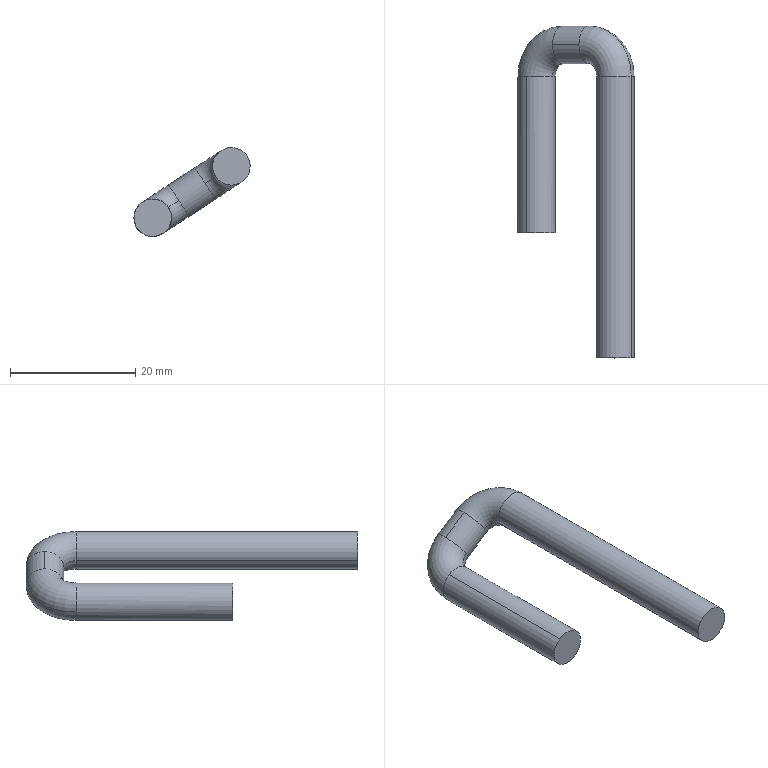Component | SolidWorks | 75-02-24RotatingHook-1 | 1 solid | 12 faces | box 18.56 x 53 x 14.2 mm | volume 2565 mm3 | cylinder 6 | torus 4 | plane 2 | commonest cylinder face diameters 6 x6 | material A3 Steel
build123d program:
from build123d import *

# Parameters (mm, degrees)
SWEEP1_PROFILE_R = 3


with BuildPart() as part:
    # Sweep1: sweep along a path in Sketch1
    with BuildLine(Plane.XY) as sweep1_path:
        Line((0, 50), (0, 5))
        ThreePointArc((0, 5), (1.464, 1.464), (5, 0))
        Line((5, 0), (10, 0))
        ThreePointArc((10, 0), (13.536, 1.464), (15, 5))
        Line((15, 5), (15, 30))
    # Sweep1 profile (on start of the path) → Sweep1 (sweep)
    with BuildSketch(Plane(origin=(0, 50, 0), x_dir=(-1, 0, 0), z_dir=(0, -1, 0))):
        Circle(SWEEP1_PROFILE_R)
    sweep(path=sweep1_path.line)


solid = part.part

# Placed as in the assembly
solid = solid.moved(Location((-17.87, 315.857, -43.68), (0, -33.158, -180)))
STEP:
#1=COLOUR_RGB('',0.7922,0.8196,0.9333);
#2=FILL_AREA_STYLE_COLOUR('',#1);
#3=FILL_AREA_STYLE('',(#2));
#4=SURFACE_STYLE_FILL_AREA(#3);
#5=SURFACE_SIDE_STYLE('',(#4));
#6=SURFACE_STYLE_USAGE(.BOTH.,#5);
#7=PRESENTATION_STYLE_ASSIGNMENT((#6));
#8=CARTESIAN_POINT('',(-1.033,12.553,-1.935));
#9=VERTEX_POINT('',#8);
#10=CARTESIAN_POINT('',(-1.098,12.435,-1.836));
#11=VERTEX_POINT('',#10);
#12=CARTESIAN_POINT('',(-1.033,12.435,-1.935));
#13=DIRECTION('',(0.8372,-0.,0.5469));
#14=DIRECTION('',(0.5469,0.,-0.8372));
#15=AXIS2_PLACEMENT_3D('',#12,#13,#14);
#16=CIRCLE('',#15,0.1181);
#17=EDGE_CURVE('',#9,#11,#16,.T.);
#18=ORIENTED_EDGE('',*,*,#17,.F.);
#19=CARTESIAN_POINT('',(-1.297,12.238,-2.107));
#20=VERTEX_POINT('',#19);
#21=CARTESIAN_POINT('',(-1.033,12.238,-1.935));
#22=DIRECTION('',(-0.5469,-0.,0.8372));
#23=DIRECTION('',(0.8372,0.,0.5469));
#24=AXIS2_PLACEMENT_3D('',#21,#22,#23);
#25=CIRCLE('',#24,0.315);
#26=EDGE_CURVE('',#9,#20,#25,.T.);
#27=ORIENTED_EDGE('',*,*,#26,.T.);
#28=CARTESIAN_POINT('',(-1.263,12.238,-1.944));
#29=VERTEX_POINT('',#28);
#30=CARTESIAN_POINT('',(-1.198,12.238,-2.043));
#31=DIRECTION('',(-0.,1.,0.));
#32=DIRECTION('',(0.5469,0.,-0.8372));
#33=AXIS2_PLACEMENT_3D('',#30,#31,#32);
#34=CIRCLE('',#33,0.1181);
#35=EDGE_CURVE('',#20,#29,#34,.T.);
#36=ORIENTED_EDGE('',*,*,#35,.T.);
#37=CARTESIAN_POINT('',(-1.099,12.238,-1.978));
#38=VERTEX_POINT('',#37);
#39=CARTESIAN_POINT('',(-1.198,12.238,-2.043));
#40=DIRECTION('',(-0.,1.,0.));
#41=DIRECTION('',(0.5469,0.,-0.8372));
#42=AXIS2_PLACEMENT_3D('',#39,#40,#41);
#43=CIRCLE('',#42,0.1181);
#44=EDGE_CURVE('',#29,#38,#43,.T.);
#45=ORIENTED_EDGE('',*,*,#44,.T.);
#46=CARTESIAN_POINT('',(-1.033,12.317,-1.935));
#47=VERTEX_POINT('',#46);
#48=CARTESIAN_POINT('',(-1.033,12.238,-1.935));
#49=DIRECTION('',(-0.5469,-0.,0.8372));
#50=DIRECTION('',(0.8372,0.,0.5469));
#51=AXIS2_PLACEMENT_3D('',#48,#49,#50);
#52=CIRCLE('',#51,0.07874);
#53=EDGE_CURVE('',#47,#38,#52,.T.);
#54=ORIENTED_EDGE('',*,*,#53,.F.);
#55=CARTESIAN_POINT('',(-1.033,12.435,-1.935));
#56=DIRECTION('',(0.8372,-0.,0.5469));
#57=DIRECTION('',(0.5469,0.,-0.8372));
#58=AXIS2_PLACEMENT_3D('',#55,#56,#57);
#59=CIRCLE('',#58,0.1181);
#60=EDGE_CURVE('',#11,#47,#59,.T.);
#61=ORIENTED_EDGE('',*,*,#60,.F.);
#62=EDGE_LOOP('',(#18,#27,#36,#45,#54,#61));
#63=FACE_OUTER_BOUND('',#62,.T.);
#64=CARTESIAN_POINT('',(-1.033,12.238,-1.935));
#65=DIRECTION('',(-0.5469,-0.,0.8372));
#66=DIRECTION('',(-0.8372,0.,-0.5469));
#67=AXIS2_PLACEMENT_3D('',#64,#65,#66);
#68=TOROIDAL_SURFACE('',#67,0.1969,0.1181);
#69=ADVANCED_FACE('',(#63),#68,.T.);
#70=CARTESIAN_POINT('',(-0.6047,12.238,-1.655));
#71=VERTEX_POINT('',#70);
#72=CARTESIAN_POINT('',(-0.8024,12.238,-1.784));
#73=VERTEX_POINT('',#72);
#74=CARTESIAN_POINT('',(-0.7036,12.238,-1.72));
#75=DIRECTION('',(-0.,-1.,-0.));
#76=DIRECTION('',(0.5469,0.,-0.8372));
#77=AXIS2_PLACEMENT_3D('',#74,#75,#76);
#78=CIRCLE('',#77,0.1181);
#79=EDGE_CURVE('',#71,#73,#78,.T.);
#80=ORIENTED_EDGE('',*,*,#79,.F.);
#81=CARTESIAN_POINT('',(-0.8684,12.553,-1.827));
#82=VERTEX_POINT('',#81);
#83=CARTESIAN_POINT('',(-0.8684,12.238,-1.827));
#84=DIRECTION('',(-0.5469,-0.,0.8372));
#85=DIRECTION('',(0.8372,0.,0.5469));
#86=AXIS2_PLACEMENT_3D('',#83,#84,#85);
#87=CIRCLE('',#86,0.315);
#88=EDGE_CURVE('',#71,#82,#87,.T.);
#89=ORIENTED_EDGE('',*,*,#88,.T.);
#90=CARTESIAN_POINT('',(-0.933,12.435,-1.728));
#91=VERTEX_POINT('',#90);
#92=CARTESIAN_POINT('',(-0.8684,12.435,-1.827));
#93=DIRECTION('',(0.8372,0.,0.5469));
#94=DIRECTION('',(0.5469,0.,-0.8372));
#95=AXIS2_PLACEMENT_3D('',#92,#93,#94);
#96=CIRCLE('',#95,0.1181);
#97=EDGE_CURVE('',#82,#91,#96,.T.);
#98=ORIENTED_EDGE('',*,*,#97,.T.);
#99=CARTESIAN_POINT('',(-0.8684,12.317,-1.827));
#100=VERTEX_POINT('',#99);
#101=CARTESIAN_POINT('',(-0.8684,12.435,-1.827));
#102=DIRECTION('',(0.8372,0.,0.5469));
#103=DIRECTION('',(0.5469,0.,-0.8372));
#104=AXIS2_PLACEMENT_3D('',#101,#102,#103);
#105=CIRCLE('',#104,0.1181);
#106=EDGE_CURVE('',#91,#100,#105,.T.);
#107=ORIENTED_EDGE('',*,*,#106,.T.);
#108=CARTESIAN_POINT('',(-0.8684,12.238,-1.827));
#109=DIRECTION('',(-0.5469,-0.,0.8372));
#110=DIRECTION('',(0.8372,0.,0.5469));
#111=AXIS2_PLACEMENT_3D('',#108,#109,#110);
#112=CIRCLE('',#111,0.07874);
#113=EDGE_CURVE('',#73,#100,#112,.T.);
#114=ORIENTED_EDGE('',*,*,#113,.F.);
#115=EDGE_LOOP('',(#80,#89,#98,#107,#114));
#116=FACE_OUTER_BOUND('',#115,.T.);
#117=CARTESIAN_POINT('',(-0.8684,12.238,-1.827));
#118=DIRECTION('',(-0.5469,-0.,0.8372));
#119=DIRECTION('',(-0.8372,0.,-0.5469));
#120=AXIS2_PLACEMENT_3D('',#117,#118,#119);
#121=TOROIDAL_SURFACE('',#120,0.1969,0.1181);
#122=ADVANCED_FACE('',(#116),#121,.T.);
#123=CARTESIAN_POINT('',(-1.133,12.238,-2.142));
#124=VERTEX_POINT('',#123);
#125=CARTESIAN_POINT('',(-1.198,12.238,-2.043));
#126=DIRECTION('',(-0.,1.,0.));
#127=DIRECTION('',(0.5469,0.,-0.8372));
#128=AXIS2_PLACEMENT_3D('',#125,#126,#127);
#129=CIRCLE('',#128,0.1181);
#130=EDGE_CURVE('',#124,#20,#129,.T.);
#131=ORIENTED_EDGE('',*,*,#130,.F.);
#132=CARTESIAN_POINT('',(-1.133,11.254,-2.142));
#133=VERTEX_POINT('',#132);
#134=CARTESIAN_POINT('',(-1.133,12.238,-2.142));
#135=DIRECTION('',(0.,-1.,-0.));
#136=VECTOR('',#135,39.37);
#137=LINE('',#134,#136);
#138=EDGE_CURVE('',#124,#133,#137,.T.);
#139=ORIENTED_EDGE('',*,*,#138,.T.);
#140=CARTESIAN_POINT('',(-1.263,11.254,-1.944));
#141=VERTEX_POINT('',#140);
#142=CARTESIAN_POINT('',(-1.198,11.254,-2.043));
#143=DIRECTION('',(-0.,1.,0.));
#144=DIRECTION('',(0.5469,0.,-0.8372));
#145=AXIS2_PLACEMENT_3D('',#142,#143,#144);
#146=CIRCLE('',#145,0.1181);
#147=EDGE_CURVE('',#133,#141,#146,.T.);
#148=ORIENTED_EDGE('',*,*,#147,.T.);
#149=CARTESIAN_POINT('',(-1.263,12.238,-1.944));
#150=DIRECTION('',(0.,-1.,-0.));
#151=VECTOR('',#150,39.37);
#152=LINE('',#149,#151);
#153=EDGE_CURVE('',#29,#141,#152,.T.);
#154=ORIENTED_EDGE('',*,*,#153,.F.);
#155=ORIENTED_EDGE('',*,*,#35,.F.);
#156=EDGE_LOOP('',(#131,#139,#148,#154,#155));
#157=FACE_OUTER_BOUND('',#156,.T.);
#158=CARTESIAN_POINT('',(-1.198,12.238,-2.043));
#159=DIRECTION('',(0.,-1.,-0.));
#160=DIRECTION('',(-0.5469,0.,0.8372));
#161=AXIS2_PLACEMENT_3D('',#158,#159,#160);
#162=CYLINDRICAL_SURFACE('',#161,0.1181);
#163=ADVANCED_FACE('',(#157),#162,.T.);
#164=ORIENTED_EDGE('',*,*,#106,.F.);
#165=CARTESIAN_POINT('',(-0.933,12.435,-1.728));
#166=DIRECTION('',(-0.8372,0.,-0.5469));
#167=VECTOR('',#166,39.37);
#168=LINE('',#165,#167);
#169=EDGE_CURVE('',#91,#11,#168,.T.);
#170=ORIENTED_EDGE('',*,*,#169,.T.);
#171=ORIENTED_EDGE('',*,*,#60,.T.);
#172=CARTESIAN_POINT('',(-0.9686,12.435,-2.034));
#173=VERTEX_POINT('',#172);
#174=CARTESIAN_POINT('',(-1.033,12.435,-1.935));
#175=DIRECTION('',(0.8372,-0.,0.5469));
#176=DIRECTION('',(0.5469,0.,-0.8372));
#177=AXIS2_PLACEMENT_3D('',#174,#175,#176);
#178=CIRCLE('',#177,0.1181);
#179=EDGE_CURVE('',#47,#173,#178,.T.);
#180=ORIENTED_EDGE('',*,*,#179,.T.);
#181=CARTESIAN_POINT('',(-0.8038,12.435,-1.926));
#182=VERTEX_POINT('',#181);
#183=CARTESIAN_POINT('',(-0.8038,12.435,-1.926));
#184=DIRECTION('',(-0.8372,0.,-0.5469));
#185=VECTOR('',#184,39.37);
#186=LINE('',#183,#185);
#187=EDGE_CURVE('',#182,#173,#186,.T.);
#188=ORIENTED_EDGE('',*,*,#187,.F.);
#189=CARTESIAN_POINT('',(-0.8684,12.435,-1.827));
#190=DIRECTION('',(0.8372,0.,0.5469));
#191=DIRECTION('',(0.5469,0.,-0.8372));
#192=AXIS2_PLACEMENT_3D('',#189,#190,#191);
#193=CIRCLE('',#192,0.1181);
#194=EDGE_CURVE('',#100,#182,#193,.T.);
#195=ORIENTED_EDGE('',*,*,#194,.F.);
#196=EDGE_LOOP('',(#164,#170,#171,#180,#188,#195));
#197=FACE_OUTER_BOUND('',#196,.T.);
#198=CARTESIAN_POINT('',(-0.8684,12.435,-1.827));
#199=DIRECTION('',(-0.8372,0.,-0.5469));
#200=DIRECTION('',(0.5469,0.,-0.8372));
#201=AXIS2_PLACEMENT_3D('',#198,#199,#200);
#202=CYLINDRICAL_SURFACE('',#201,0.1181);
#203=ADVANCED_FACE('',(#197),#202,.T.);
#204=CARTESIAN_POINT('',(-0.6047,10.467,-1.655));
#205=VERTEX_POINT('',#204);
#206=CARTESIAN_POINT('',(-0.8024,10.467,-1.784));
#207=VERTEX_POINT('',#206);
#208=CARTESIAN_POINT('',(-0.7036,10.467,-1.72));
#209=DIRECTION('',(-0.,-1.,-0.));
#210=DIRECTION('',(0.5469,0.,-0.8372));
#211=AXIS2_PLACEMENT_3D('',#208,#209,#210);
#212=CIRCLE('',#211,0.1181);
#213=EDGE_CURVE('',#205,#207,#212,.T.);
#214=ORIENTED_EDGE('',*,*,#213,.F.);
#215=CARTESIAN_POINT('',(-0.6047,10.467,-1.655));
#216=DIRECTION('',(0.,1.,0.));
#217=VECTOR('',#216,39.37);
#218=LINE('',#215,#217);
#219=EDGE_CURVE('',#205,#71,#218,.T.);
#220=ORIENTED_EDGE('',*,*,#219,.T.);
#221=ORIENTED_EDGE('',*,*,#79,.T.);
#222=CARTESIAN_POINT('',(-0.8024,10.467,-1.784));
#223=DIRECTION('',(0.,1.,0.));
#224=VECTOR('',#223,39.37);
#225=LINE('',#222,#224);
#226=EDGE_CURVE('',#207,#73,#225,.T.);
#227=ORIENTED_EDGE('',*,*,#226,.F.);
#228=EDGE_LOOP('',(#214,#220,#221,#227));
#229=FACE_OUTER_BOUND('',#228,.T.);
#230=CARTESIAN_POINT('',(-0.7036,10.467,-1.72));
#231=DIRECTION('',(0.,1.,0.));
#232=DIRECTION('',(-0.8372,0.,-0.5469));
#233=AXIS2_PLACEMENT_3D('',#230,#231,#232);
#234=CYLINDRICAL_SURFACE('',#233,0.1181);
#235=ADVANCED_FACE('',(#229),#234,.T.);
#236=ORIENTED_EDGE('',*,*,#138,.F.);
#237=CARTESIAN_POINT('',(-1.198,12.238,-2.043));
#238=DIRECTION('',(-0.,1.,0.));
#239=DIRECTION('',(0.5469,0.,-0.8372));
#240=AXIS2_PLACEMENT_3D('',#237,#238,#239);
#241=CIRCLE('',#240,0.1181);
#242=EDGE_CURVE('',#38,#124,#241,.T.);
#243=ORIENTED_EDGE('',*,*,#242,.F.);
#244=ORIENTED_EDGE('',*,*,#44,.F.);
#245=ORIENTED_EDGE('',*,*,#153,.T.);
#246=CARTESIAN_POINT('',(-1.198,11.254,-2.043));
#247=DIRECTION('',(-0.,1.,0.));
#248=DIRECTION('',(0.5469,0.,-0.8372));
#249=AXIS2_PLACEMENT_3D('',#246,#247,#248);
#250=CIRCLE('',#249,0.1181);
#251=EDGE_CURVE('',#141,#133,#250,.T.);
#252=ORIENTED_EDGE('',*,*,#251,.T.);
#253=EDGE_LOOP('',(#236,#243,#244,#245,#252));
#254=FACE_OUTER_BOUND('',#253,.T.);
#255=CARTESIAN_POINT('',(-1.198,12.238,-2.043));
#256=DIRECTION('',(0.,-1.,-0.));
#257=DIRECTION('',(-0.5469,0.,0.8372));
#258=AXIS2_PLACEMENT_3D('',#255,#256,#257);
#259=CYLINDRICAL_SURFACE('',#258,0.1181);
#260=ADVANCED_FACE('',(#254),#259,.T.);
#261=ORIENTED_EDGE('',*,*,#26,.F.);
#262=CARTESIAN_POINT('',(-1.033,12.435,-1.935));
#263=DIRECTION('',(0.8372,-0.,0.5469));
#264=DIRECTION('',(0.5469,0.,-0.8372));
#265=AXIS2_PLACEMENT_3D('',#262,#263,#264);
#266=CIRCLE('',#265,0.1181);
#267=EDGE_CURVE('',#173,#9,#266,.T.);
#268=ORIENTED_EDGE('',*,*,#267,.F.);
#269=ORIENTED_EDGE('',*,*,#179,.F.);
#270=ORIENTED_EDGE('',*,*,#53,.T.);
#271=ORIENTED_EDGE('',*,*,#242,.T.);
#272=ORIENTED_EDGE('',*,*,#130,.T.);
#273=EDGE_LOOP('',(#261,#268,#269,#270,#271,#272));
#274=FACE_OUTER_BOUND('',#273,.T.);
#275=CARTESIAN_POINT('',(-1.033,12.238,-1.935));
#276=DIRECTION('',(-0.5469,-0.,0.8372));
#277=DIRECTION('',(-0.8372,0.,-0.5469));
#278=AXIS2_PLACEMENT_3D('',#275,#276,#277);
#279=TOROIDAL_SURFACE('',#278,0.1969,0.1181);
#280=ADVANCED_FACE('',(#274),#279,.T.);
#281=ORIENTED_EDGE('',*,*,#169,.F.);
#282=ORIENTED_EDGE('',*,*,#97,.F.);
#283=CARTESIAN_POINT('',(-0.8684,12.435,-1.827));
#284=DIRECTION('',(0.8372,0.,0.5469));
#285=DIRECTION('',(0.5469,0.,-0.8372));
#286=AXIS2_PLACEMENT_3D('',#283,#284,#285);
#287=CIRCLE('',#286,0.1181);
#288=EDGE_CURVE('',#182,#82,#287,.T.);
#289=ORIENTED_EDGE('',*,*,#288,.F.);
#290=ORIENTED_EDGE('',*,*,#187,.T.);
#291=ORIENTED_EDGE('',*,*,#267,.T.);
#292=ORIENTED_EDGE('',*,*,#17,.T.);
#293=EDGE_LOOP('',(#281,#282,#289,#290,#291,#292));
#294=FACE_OUTER_BOUND('',#293,.T.);
#295=CARTESIAN_POINT('',(-0.8684,12.435,-1.827));
#296=DIRECTION('',(-0.8372,0.,-0.5469));
#297=DIRECTION('',(0.5469,0.,-0.8372));
#298=AXIS2_PLACEMENT_3D('',#295,#296,#297);
#299=CYLINDRICAL_SURFACE('',#298,0.1181);
#300=ADVANCED_FACE('',(#294),#299,.T.);
#301=ORIENTED_EDGE('',*,*,#88,.F.);
#302=CARTESIAN_POINT('',(-0.7036,12.238,-1.72));
#303=DIRECTION('',(-0.,-1.,-0.));
#304=DIRECTION('',(0.5469,0.,-0.8372));
#305=AXIS2_PLACEMENT_3D('',#302,#303,#304);
#306=CIRCLE('',#305,0.1181);
#307=EDGE_CURVE('',#73,#71,#306,.T.);
#308=ORIENTED_EDGE('',*,*,#307,.F.);
#309=ORIENTED_EDGE('',*,*,#113,.T.);
#310=ORIENTED_EDGE('',*,*,#194,.T.);
#311=ORIENTED_EDGE('',*,*,#288,.T.);
#312=EDGE_LOOP('',(#301,#308,#309,#310,#311));
#313=FACE_OUTER_BOUND('',#312,.T.);
#314=CARTESIAN_POINT('',(-0.8684,12.238,-1.827));
#315=DIRECTION('',(-0.5469,-0.,0.8372));
#316=DIRECTION('',(-0.8372,0.,-0.5469));
#317=AXIS2_PLACEMENT_3D('',#314,#315,#316);
#318=TOROIDAL_SURFACE('',#317,0.1969,0.1181);
#319=ADVANCED_FACE('',(#313),#318,.T.);
#320=ORIENTED_EDGE('',*,*,#219,.F.);
#321=CARTESIAN_POINT('',(-0.7036,10.467,-1.72));
#322=DIRECTION('',(-0.,-1.,-0.));
#323=DIRECTION('',(0.5469,0.,-0.8372));
#324=AXIS2_PLACEMENT_3D('',#321,#322,#323);
#325=CIRCLE('',#324,0.1181);
#326=EDGE_CURVE('',#207,#205,#325,.T.);
#327=ORIENTED_EDGE('',*,*,#326,.F.);
#328=ORIENTED_EDGE('',*,*,#226,.T.);
#329=ORIENTED_EDGE('',*,*,#307,.T.);
#330=EDGE_LOOP('',(#320,#327,#328,#329));
#331=FACE_OUTER_BOUND('',#330,.T.);
#332=CARTESIAN_POINT('',(-0.7036,10.467,-1.72));
#333=DIRECTION('',(0.,1.,0.));
#334=DIRECTION('',(-0.8372,0.,-0.5469));
#335=AXIS2_PLACEMENT_3D('',#332,#333,#334);
#336=CYLINDRICAL_SURFACE('',#335,0.1181);
#337=ADVANCED_FACE('',(#331),#336,.T.);
#338=ORIENTED_EDGE('',*,*,#251,.F.);
#339=ORIENTED_EDGE('',*,*,#147,.F.);
#340=EDGE_LOOP('',(#338,#339));
#341=FACE_OUTER_BOUND('',#340,.T.);
#342=CARTESIAN_POINT('',(-1.198,11.254,-2.043));
#343=DIRECTION('',(-0.,1.,0.));
#344=DIRECTION('',(0.5469,0.,-0.8372));
#345=AXIS2_PLACEMENT_3D('',#342,#343,#344);
#346=PLANE('',#345);
#347=ADVANCED_FACE('',(#341),#346,.F.);
#348=ORIENTED_EDGE('',*,*,#326,.T.);
#349=ORIENTED_EDGE('',*,*,#213,.T.);
#350=EDGE_LOOP('',(#348,#349));
#351=FACE_OUTER_BOUND('',#350,.T.);
#352=CARTESIAN_POINT('',(-0.7036,10.467,-1.72));
#353=DIRECTION('',(-0.,-1.,-0.));
#354=DIRECTION('',(0.5469,0.,-0.8372));
#355=AXIS2_PLACEMENT_3D('',#352,#353,#354);
#356=PLANE('',#355);
#357=ADVANCED_FACE('',(#351),#356,.T.);
#358=CLOSED_SHELL('',(#69,#122,#163,#203,#235,#260,#280,#300,#319,#337,#347,#357));
#359=MANIFOLD_SOLID_BREP('',#358);
#360=STYLED_ITEM('',(#7),#359);
#361=(LENGTH_UNIT()NAMED_UNIT(*)SI_UNIT($,.METRE.));
#362=LENGTH_MEASURE_WITH_UNIT(LENGTH_MEASURE(0.0254),#361);
#363=DIMENSIONAL_EXPONENTS(1.,0.,0.,0.,0.,0.,0.);
#364=(CONVERSION_BASED_UNIT('',#362)LENGTH_UNIT()NAMED_UNIT(#363));
#365=UNCERTAINTY_MEASURE_WITH_UNIT(LENGTH_MEASURE(0.00001),#364,'','');
#366=(NAMED_UNIT(*)PLANE_ANGLE_UNIT()SI_UNIT($,.RADIAN.));
#367=(NAMED_UNIT(*)SI_UNIT($,.STERADIAN.)SOLID_ANGLE_UNIT());
#368=(GEOMETRIC_REPRESENTATION_CONTEXT(3)GLOBAL_UNCERTAINTY_ASSIGNED_CONTEXT((#365))GLOBAL_UNIT_ASSIGNED_CONTEXT((#364,#366,#367))REPRESENTATION_CONTEXT('',''));
#369=MECHANICAL_DESIGN_GEOMETRIC_PRESENTATION_REPRESENTATION('',(#360),#368);
#370=CARTESIAN_POINT('',(0.,0.,0.));
#371=DIRECTION('',(0.,0.,1.));
#372=DIRECTION('',(1.,0.,0.));
#373=AXIS2_PLACEMENT_3D('',#370,#371,#372);
#374=(LENGTH_UNIT()NAMED_UNIT(*)SI_UNIT($,.METRE.));
#375=LENGTH_MEASURE_WITH_UNIT(LENGTH_MEASURE(0.0254),#374);
#376=DIMENSIONAL_EXPONENTS(1.,0.,0.,0.,0.,0.,0.);
#377=(CONVERSION_BASED_UNIT('',#375)LENGTH_UNIT()NAMED_UNIT(#376));
#378=UNCERTAINTY_MEASURE_WITH_UNIT(LENGTH_MEASURE(0.00001),#377,'','');
#379=(NAMED_UNIT(*)PLANE_ANGLE_UNIT()SI_UNIT($,.RADIAN.));
#380=(NAMED_UNIT(*)SI_UNIT($,.STERADIAN.)SOLID_ANGLE_UNIT());
#381=(GEOMETRIC_REPRESENTATION_CONTEXT(3)GLOBAL_UNCERTAINTY_ASSIGNED_CONTEXT((#378))GLOBAL_UNIT_ASSIGNED_CONTEXT((#377,#379,#380))REPRESENTATION_CONTEXT('',''));
#382=ADVANCED_BREP_SHAPE_REPRESENTATION('',(#359,#373),#381);
#383=PRESENTATION_LAYER_ASSIGNMENT('','',(#360));